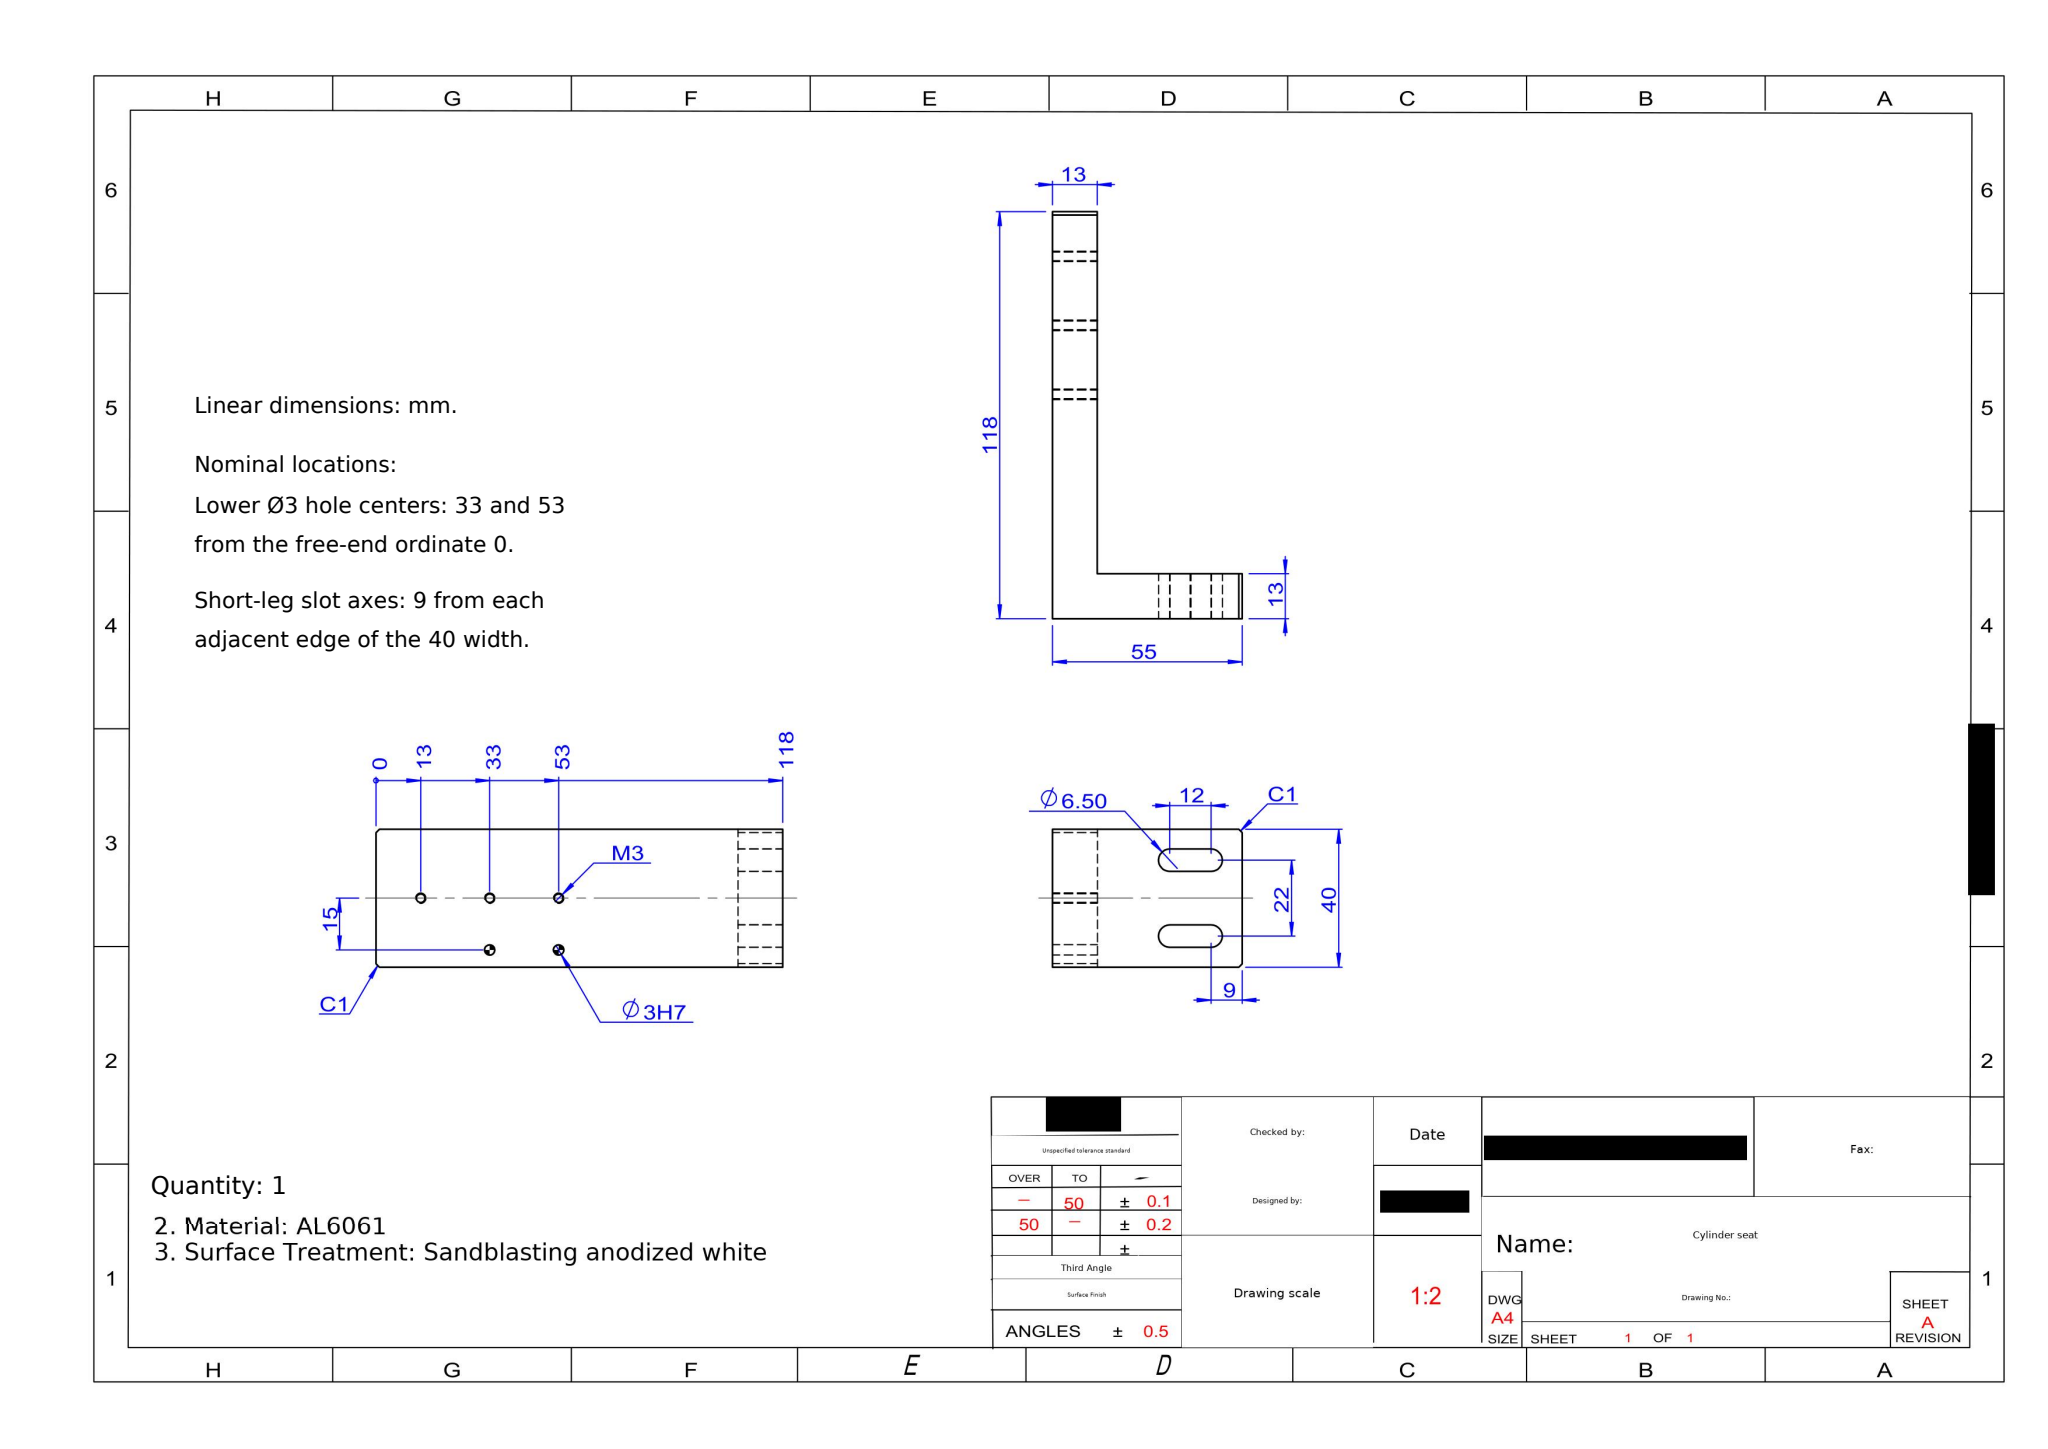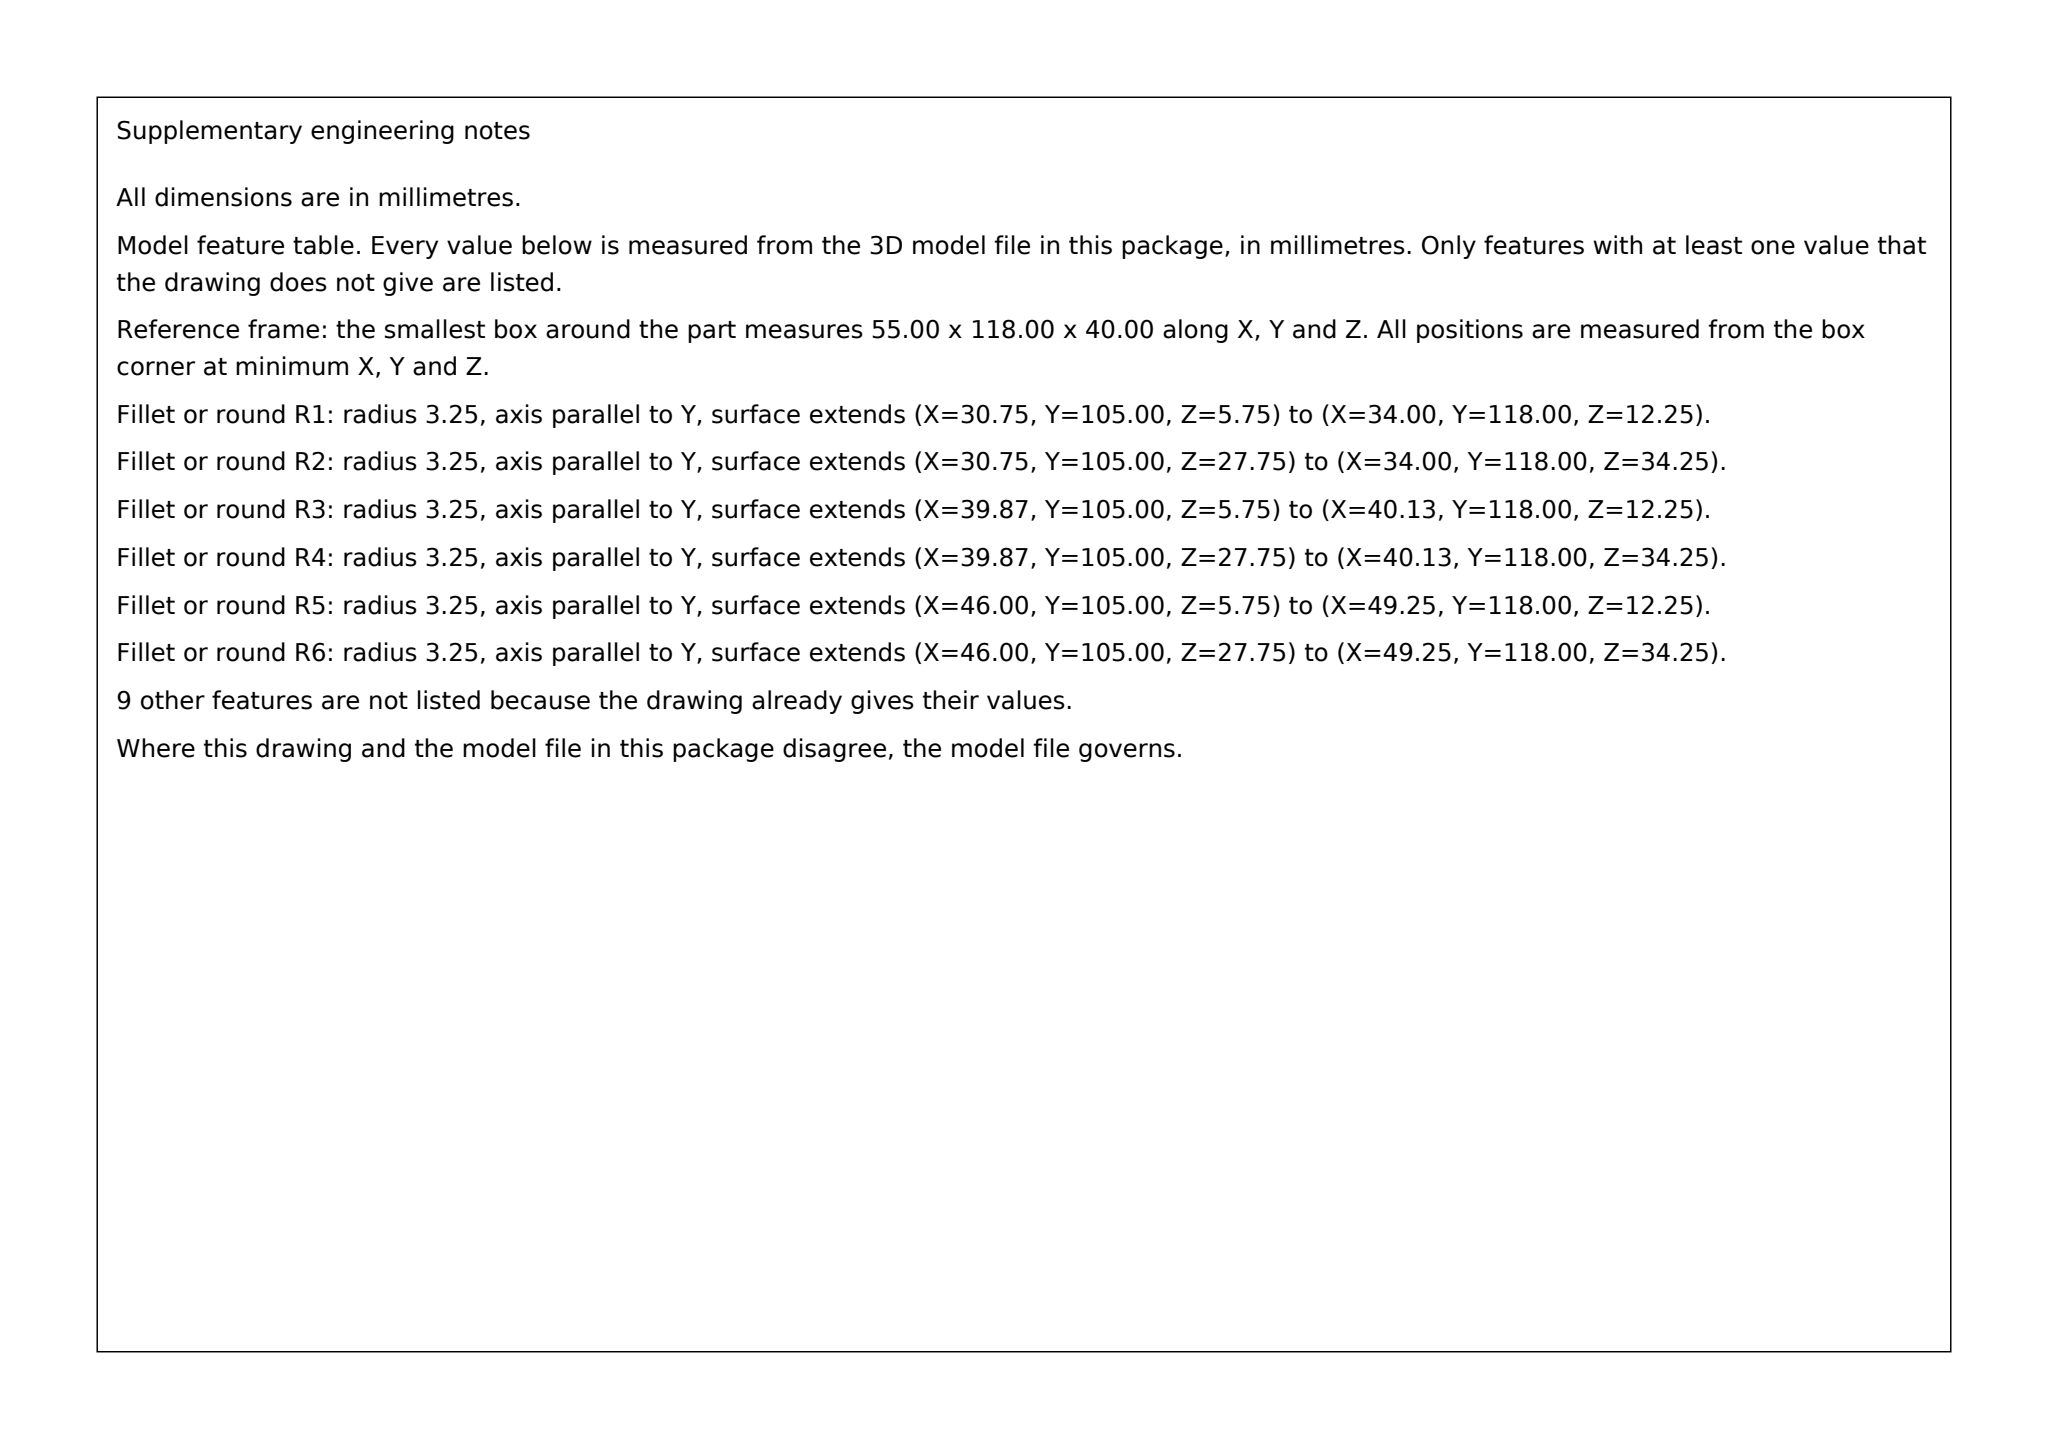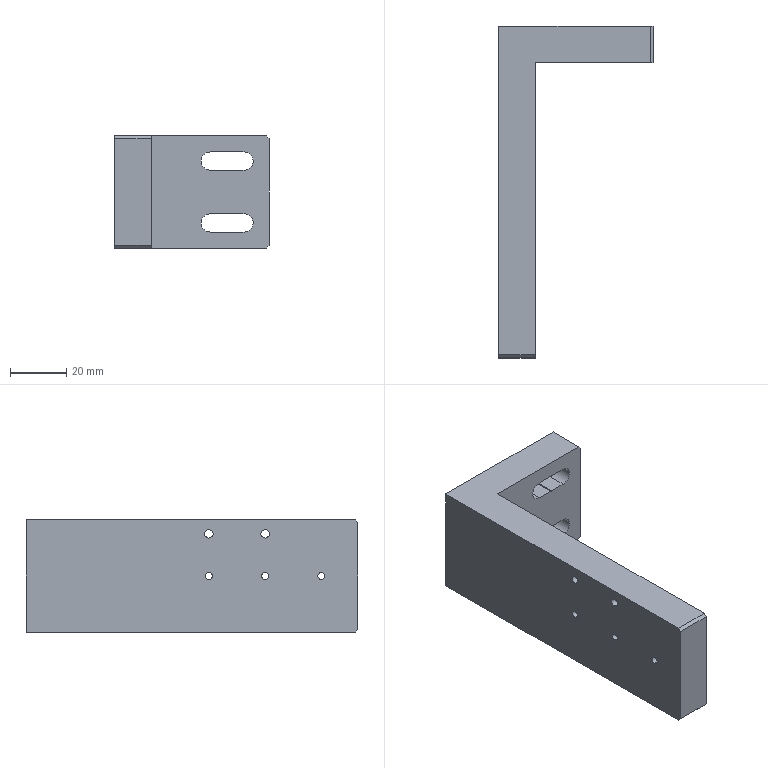Part | SolidWorks | mm | material AL6061 | 1 solid | 40 faces | box 55 x 118 x 40 mm | volume 79911 mm3 | cylinder 20 | plane 20 | commonest cylinder face diameters 2.5 x6 6.495 x6 3 x4 6.5 x4